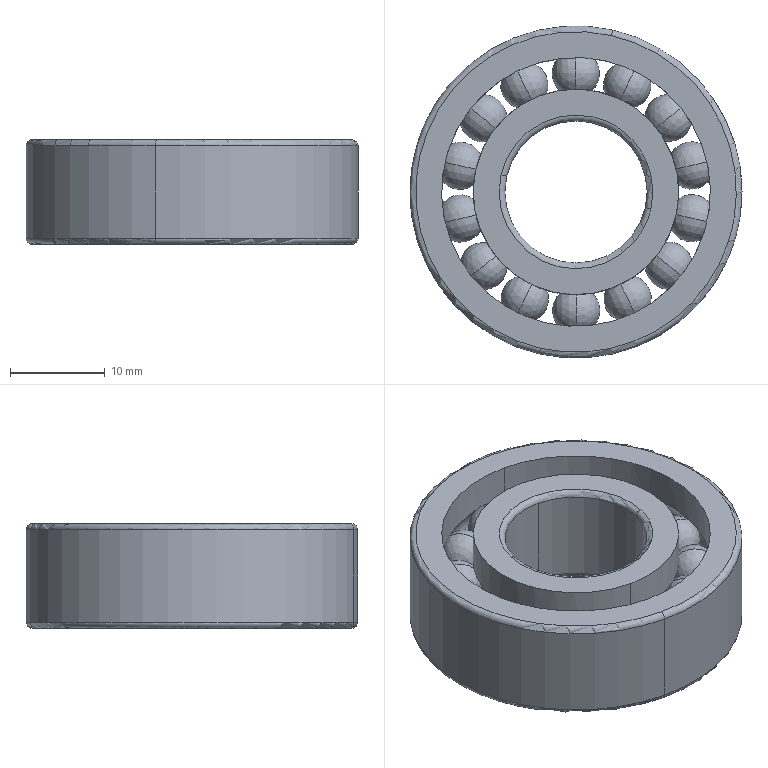Component | SolidWorks | DoubleFilmTransport-1_DeepGrooveBallBearing6202_DeepGrooveBallBearing6202-2 | 1 solid | 97 faces | volume 6333 mm3 | torus 53 | sphere 28 | cylinder 12 | plane 4 | commonest cylinder face diameters 28.333 x4 21.667 x4 35 x2 15 x2